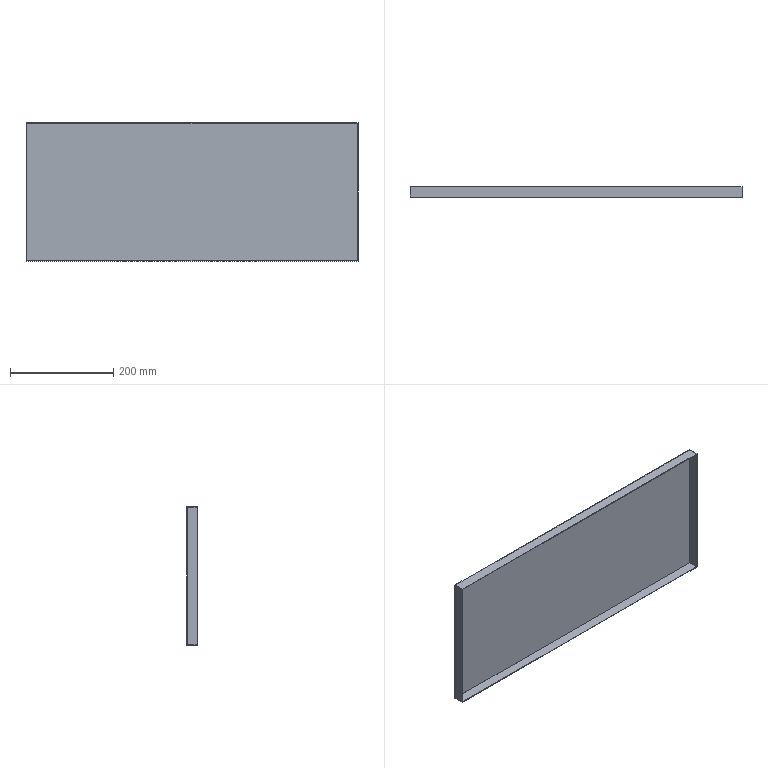Component | SolidWorks | FrameAssembly-1_FrameWeldment-1_BottomThinPlate-1 | 1 solid | 11 faces | box 644 x 20 x 269 mm | volume 248969 mm3 | plane 11
build123d program:
from build123d import *

# Parameters (mm, degrees)
SKETCH1_W           = 644
SKETCH1_H           = 269
BOSS_EXTRUDE1_DEPTH = 20
SKETCH2_W           = 641.6
SKETCH2_H           = 266.6
CUT_EXTRUDE1_DEPTH  = 18.8


with BuildPart() as part:
    # Sketch1 → Boss-Extrude1 (new body)
    with BuildSketch(Plane(origin=(0, 0, 0), x_dir=(-1, 0, 0), z_dir=(0, 0, -1))):
        Rectangle(SKETCH1_W, SKETCH1_H)
    extrude(amount=-BOSS_EXTRUDE1_DEPTH)

    # Sketch2 → Cut-Extrude1 (cut)
    with BuildSketch(Plane(origin=(0, 0, 0), x_dir=(-1, 0, 0), z_dir=(0, 0, -1))):
        Rectangle(SKETCH2_W, SKETCH2_H)
    extrude(amount=-CUT_EXTRUDE1_DEPTH, mode=Mode.SUBTRACT)


solid = part.part

# Placed as in the assembly
solid = solid.moved(Location((-298.746, -418.627, -192), (-90, 0, 0)))
STEP:
#1=COLOUR_RGB('',0.7922,0.8196,0.9333);
#2=FILL_AREA_STYLE_COLOUR('',#1);
#3=FILL_AREA_STYLE('',(#2));
#4=SURFACE_STYLE_FILL_AREA(#3);
#5=SURFACE_SIDE_STYLE('',(#4));
#6=SURFACE_STYLE_USAGE(.BOTH.,#5);
#7=PRESENTATION_STYLE_ASSIGNMENT((#6));
#8=CARTESIAN_POINT('',(0.9155,-16.481,-2.264));
#9=VERTEX_POINT('',#8);
#10=CARTESIAN_POINT('',(-24.439,-16.481,-2.264));
#11=VERTEX_POINT('',#10);
#12=CARTESIAN_POINT('',(0.9155,-16.481,-2.264));
#13=DIRECTION('',(-1.,0.,0.));
#14=VECTOR('',#13,39.37);
#15=LINE('',#12,#14);
#16=EDGE_CURVE('',#9,#11,#15,.T.);
#17=ORIENTED_EDGE('',*,*,#16,.F.);
#18=CARTESIAN_POINT('',(0.9155,-15.694,-2.264));
#19=VERTEX_POINT('',#18);
#20=CARTESIAN_POINT('',(0.9155,-15.694,-2.264));
#21=DIRECTION('',(-0.,-1.,0.));
#22=VECTOR('',#21,39.37);
#23=LINE('',#20,#22);
#24=EDGE_CURVE('',#19,#9,#23,.T.);
#25=ORIENTED_EDGE('',*,*,#24,.F.);
#26=CARTESIAN_POINT('',(-24.439,-15.694,-2.264));
#27=VERTEX_POINT('',#26);
#28=CARTESIAN_POINT('',(0.9155,-15.694,-2.264));
#29=DIRECTION('',(-1.,0.,0.));
#30=VECTOR('',#29,39.37);
#31=LINE('',#28,#30);
#32=EDGE_CURVE('',#19,#27,#31,.T.);
#33=ORIENTED_EDGE('',*,*,#32,.T.);
#34=CARTESIAN_POINT('',(-24.439,-15.694,-2.264));
#35=DIRECTION('',(-0.,-1.,0.));
#36=VECTOR('',#35,39.37);
#37=LINE('',#34,#36);
#38=EDGE_CURVE('',#27,#11,#37,.T.);
#39=ORIENTED_EDGE('',*,*,#38,.T.);
#40=EDGE_LOOP('',(#17,#25,#33,#39));
#41=FACE_OUTER_BOUND('',#40,.T.);
#42=CARTESIAN_POINT('',(0.9155,-15.694,-2.264));
#43=DIRECTION('',(0.,0.,1.));
#44=DIRECTION('',(-0.,-1.,0.));
#45=AXIS2_PLACEMENT_3D('',#42,#43,#44);
#46=PLANE('',#45);
#47=ADVANCED_FACE('',(#41),#46,.T.);
#48=CARTESIAN_POINT('',(0.9155,-16.481,-12.854));
#49=VERTEX_POINT('',#48);
#50=CARTESIAN_POINT('',(0.9155,-16.481,-12.854));
#51=DIRECTION('',(-0.,0.,1.));
#52=VECTOR('',#51,39.37);
#53=LINE('',#50,#52);
#54=EDGE_CURVE('',#49,#9,#53,.T.);
#55=ORIENTED_EDGE('',*,*,#54,.F.);
#56=CARTESIAN_POINT('',(0.9155,-15.694,-12.854));
#57=VERTEX_POINT('',#56);
#58=CARTESIAN_POINT('',(0.9155,-15.694,-12.854));
#59=DIRECTION('',(-0.,-1.,0.));
#60=VECTOR('',#59,39.37);
#61=LINE('',#58,#60);
#62=EDGE_CURVE('',#57,#49,#61,.T.);
#63=ORIENTED_EDGE('',*,*,#62,.F.);
#64=CARTESIAN_POINT('',(0.9155,-15.694,-12.854));
#65=DIRECTION('',(-0.,0.,1.));
#66=VECTOR('',#65,39.37);
#67=LINE('',#64,#66);
#68=EDGE_CURVE('',#57,#19,#67,.T.);
#69=ORIENTED_EDGE('',*,*,#68,.T.);
#70=ORIENTED_EDGE('',*,*,#24,.T.);
#71=EDGE_LOOP('',(#55,#63,#69,#70));
#72=FACE_OUTER_BOUND('',#71,.T.);
#73=CARTESIAN_POINT('',(0.9155,-15.694,-12.854));
#74=DIRECTION('',(1.,-0.,0.));
#75=DIRECTION('',(0.,-0.,-1.));
#76=AXIS2_PLACEMENT_3D('',#73,#74,#75);
#77=PLANE('',#76);
#78=ADVANCED_FACE('',(#72),#77,.T.);
#79=CARTESIAN_POINT('',(-24.439,-16.481,-12.854));
#80=VERTEX_POINT('',#79);
#81=CARTESIAN_POINT('',(-24.439,-16.481,-12.854));
#82=DIRECTION('',(1.,-0.,0.));
#83=VECTOR('',#82,39.37);
#84=LINE('',#81,#83);
#85=EDGE_CURVE('',#80,#49,#84,.T.);
#86=ORIENTED_EDGE('',*,*,#85,.F.);
#87=CARTESIAN_POINT('',(-24.439,-15.694,-12.854));
#88=VERTEX_POINT('',#87);
#89=CARTESIAN_POINT('',(-24.439,-15.694,-12.854));
#90=DIRECTION('',(-0.,-1.,0.));
#91=VECTOR('',#90,39.37);
#92=LINE('',#89,#91);
#93=EDGE_CURVE('',#88,#80,#92,.T.);
#94=ORIENTED_EDGE('',*,*,#93,.F.);
#95=CARTESIAN_POINT('',(-24.439,-15.694,-12.854));
#96=DIRECTION('',(1.,-0.,0.));
#97=VECTOR('',#96,39.37);
#98=LINE('',#95,#97);
#99=EDGE_CURVE('',#88,#57,#98,.T.);
#100=ORIENTED_EDGE('',*,*,#99,.T.);
#101=ORIENTED_EDGE('',*,*,#62,.T.);
#102=EDGE_LOOP('',(#86,#94,#100,#101));
#103=FACE_OUTER_BOUND('',#102,.T.);
#104=CARTESIAN_POINT('',(-24.439,-15.694,-12.854));
#105=DIRECTION('',(-0.,-0.,-1.));
#106=DIRECTION('',(0.,1.,-0.));
#107=AXIS2_PLACEMENT_3D('',#104,#105,#106);
#108=PLANE('',#107);
#109=ADVANCED_FACE('',(#103),#108,.T.);
#110=CARTESIAN_POINT('',(-24.439,-16.481,-2.264));
#111=DIRECTION('',(-0.,0.,-1.));
#112=VECTOR('',#111,39.37);
#113=LINE('',#110,#112);
#114=EDGE_CURVE('',#11,#80,#113,.T.);
#115=ORIENTED_EDGE('',*,*,#114,.F.);
#116=ORIENTED_EDGE('',*,*,#38,.F.);
#117=CARTESIAN_POINT('',(-24.439,-15.694,-2.264));
#118=DIRECTION('',(-0.,0.,-1.));
#119=VECTOR('',#118,39.37);
#120=LINE('',#117,#119);
#121=EDGE_CURVE('',#27,#88,#120,.T.);
#122=ORIENTED_EDGE('',*,*,#121,.T.);
#123=ORIENTED_EDGE('',*,*,#93,.T.);
#124=EDGE_LOOP('',(#115,#116,#122,#123));
#125=FACE_OUTER_BOUND('',#124,.T.);
#126=CARTESIAN_POINT('',(-24.439,-15.694,-2.264));
#127=DIRECTION('',(-1.,0.,0.));
#128=DIRECTION('',(0.,-0.,1.));
#129=AXIS2_PLACEMENT_3D('',#126,#127,#128);
#130=PLANE('',#129);
#131=ADVANCED_FACE('',(#125),#130,.T.);
#132=ORIENTED_EDGE('',*,*,#32,.F.);
#133=ORIENTED_EDGE('',*,*,#68,.F.);
#134=ORIENTED_EDGE('',*,*,#99,.F.);
#135=ORIENTED_EDGE('',*,*,#121,.F.);
#136=EDGE_LOOP('',(#132,#133,#134,#135));
#137=FACE_OUTER_BOUND('',#136,.T.);
#138=CARTESIAN_POINT('',(-11.762,-15.694,-7.559));
#139=DIRECTION('',(-0.,-1.,0.));
#140=DIRECTION('',(-1.,0.,0.));
#141=AXIS2_PLACEMENT_3D('',#138,#139,#140);
#142=PLANE('',#141);
#143=ADVANCED_FACE('',(#137),#142,.F.);
#144=CARTESIAN_POINT('',(0.8683,-16.481,-12.807));
#145=VERTEX_POINT('',#144);
#146=CARTESIAN_POINT('',(0.8683,-16.481,-2.311));
#147=VERTEX_POINT('',#146);
#148=CARTESIAN_POINT('',(0.8683,-16.481,-12.807));
#149=DIRECTION('',(0.,0.,1.));
#150=VECTOR('',#149,39.37);
#151=LINE('',#148,#150);
#152=EDGE_CURVE('',#145,#147,#151,.T.);
#153=ORIENTED_EDGE('',*,*,#152,.F.);
#154=CARTESIAN_POINT('',(-24.392,-16.481,-12.807));
#155=VERTEX_POINT('',#154);
#156=CARTESIAN_POINT('',(-24.392,-16.481,-12.807));
#157=DIRECTION('',(1.,-0.,0.));
#158=VECTOR('',#157,39.37);
#159=LINE('',#156,#158);
#160=EDGE_CURVE('',#155,#145,#159,.T.);
#161=ORIENTED_EDGE('',*,*,#160,.F.);
#162=CARTESIAN_POINT('',(-24.392,-16.481,-2.311));
#163=VERTEX_POINT('',#162);
#164=CARTESIAN_POINT('',(-24.392,-16.481,-2.311));
#165=DIRECTION('',(-0.,-0.,-1.));
#166=VECTOR('',#165,39.37);
#167=LINE('',#164,#166);
#168=EDGE_CURVE('',#163,#155,#167,.T.);
#169=ORIENTED_EDGE('',*,*,#168,.F.);
#170=CARTESIAN_POINT('',(0.8683,-16.481,-2.311));
#171=DIRECTION('',(-1.,0.,0.));
#172=VECTOR('',#171,39.37);
#173=LINE('',#170,#172);
#174=EDGE_CURVE('',#147,#163,#173,.T.);
#175=ORIENTED_EDGE('',*,*,#174,.F.);
#176=EDGE_LOOP('',(#153,#161,#169,#175));
#177=FACE_BOUND('',#176,.T.);
#178=ORIENTED_EDGE('',*,*,#16,.T.);
#179=ORIENTED_EDGE('',*,*,#114,.T.);
#180=ORIENTED_EDGE('',*,*,#85,.T.);
#181=ORIENTED_EDGE('',*,*,#54,.T.);
#182=EDGE_LOOP('',(#178,#179,#180,#181));
#183=FACE_OUTER_BOUND('',#182,.T.);
#184=CARTESIAN_POINT('',(-11.762,-16.481,-7.559));
#185=DIRECTION('',(-0.,-1.,0.));
#186=DIRECTION('',(-1.,0.,0.));
#187=AXIS2_PLACEMENT_3D('',#184,#185,#186);
#188=PLANE('',#187);
#189=ADVANCED_FACE('',(#177,#183),#188,.T.);
#190=ORIENTED_EDGE('',*,*,#152,.T.);
#191=CARTESIAN_POINT('',(0.8683,-15.741,-2.311));
#192=VERTEX_POINT('',#191);
#193=CARTESIAN_POINT('',(0.8683,-15.741,-2.311));
#194=DIRECTION('',(-0.,-1.,0.));
#195=VECTOR('',#194,39.37);
#196=LINE('',#193,#195);
#197=EDGE_CURVE('',#192,#147,#196,.T.);
#198=ORIENTED_EDGE('',*,*,#197,.F.);
#199=CARTESIAN_POINT('',(0.8683,-15.741,-12.807));
#200=VERTEX_POINT('',#199);
#201=CARTESIAN_POINT('',(0.8683,-15.741,-12.807));
#202=DIRECTION('',(0.,0.,1.));
#203=VECTOR('',#202,39.37);
#204=LINE('',#201,#203);
#205=EDGE_CURVE('',#200,#192,#204,.T.);
#206=ORIENTED_EDGE('',*,*,#205,.F.);
#207=CARTESIAN_POINT('',(0.8683,-15.741,-12.807));
#208=DIRECTION('',(-0.,-1.,0.));
#209=VECTOR('',#208,39.37);
#210=LINE('',#207,#209);
#211=EDGE_CURVE('',#200,#145,#210,.T.);
#212=ORIENTED_EDGE('',*,*,#211,.T.);
#213=EDGE_LOOP('',(#190,#198,#206,#212));
#214=FACE_OUTER_BOUND('',#213,.T.);
#215=CARTESIAN_POINT('',(0.8683,-15.741,-12.807));
#216=DIRECTION('',(1.,-0.,0.));
#217=DIRECTION('',(-0.,-1.,0.));
#218=AXIS2_PLACEMENT_3D('',#215,#216,#217);
#219=PLANE('',#218);
#220=ADVANCED_FACE('',(#214),#219,.F.);
#221=ORIENTED_EDGE('',*,*,#160,.T.);
#222=ORIENTED_EDGE('',*,*,#211,.F.);
#223=CARTESIAN_POINT('',(-24.392,-15.741,-12.807));
#224=VERTEX_POINT('',#223);
#225=CARTESIAN_POINT('',(-24.392,-15.741,-12.807));
#226=DIRECTION('',(1.,-0.,0.));
#227=VECTOR('',#226,39.37);
#228=LINE('',#225,#227);
#229=EDGE_CURVE('',#224,#200,#228,.T.);
#230=ORIENTED_EDGE('',*,*,#229,.F.);
#231=CARTESIAN_POINT('',(-24.392,-15.741,-12.807));
#232=DIRECTION('',(-0.,-1.,0.));
#233=VECTOR('',#232,39.37);
#234=LINE('',#231,#233);
#235=EDGE_CURVE('',#224,#155,#234,.T.);
#236=ORIENTED_EDGE('',*,*,#235,.T.);
#237=EDGE_LOOP('',(#221,#222,#230,#236));
#238=FACE_OUTER_BOUND('',#237,.T.);
#239=CARTESIAN_POINT('',(-24.392,-15.741,-12.807));
#240=DIRECTION('',(-0.,-0.,-1.));
#241=DIRECTION('',(0.,1.,-0.));
#242=AXIS2_PLACEMENT_3D('',#239,#240,#241);
#243=PLANE('',#242);
#244=ADVANCED_FACE('',(#238),#243,.F.);
#245=ORIENTED_EDGE('',*,*,#168,.T.);
#246=ORIENTED_EDGE('',*,*,#235,.F.);
#247=CARTESIAN_POINT('',(-24.392,-15.741,-2.311));
#248=VERTEX_POINT('',#247);
#249=CARTESIAN_POINT('',(-24.392,-15.741,-2.311));
#250=DIRECTION('',(-0.,-0.,-1.));
#251=VECTOR('',#250,39.37);
#252=LINE('',#249,#251);
#253=EDGE_CURVE('',#248,#224,#252,.T.);
#254=ORIENTED_EDGE('',*,*,#253,.F.);
#255=CARTESIAN_POINT('',(-24.392,-15.741,-2.311));
#256=DIRECTION('',(-0.,-1.,0.));
#257=VECTOR('',#256,39.37);
#258=LINE('',#255,#257);
#259=EDGE_CURVE('',#248,#163,#258,.T.);
#260=ORIENTED_EDGE('',*,*,#259,.T.);
#261=EDGE_LOOP('',(#245,#246,#254,#260));
#262=FACE_OUTER_BOUND('',#261,.T.);
#263=CARTESIAN_POINT('',(-24.392,-15.741,-2.311));
#264=DIRECTION('',(-1.,0.,-0.));
#265=DIRECTION('',(0.,1.,-0.));
#266=AXIS2_PLACEMENT_3D('',#263,#264,#265);
#267=PLANE('',#266);
#268=ADVANCED_FACE('',(#262),#267,.F.);
#269=ORIENTED_EDGE('',*,*,#174,.T.);
#270=ORIENTED_EDGE('',*,*,#259,.F.);
#271=CARTESIAN_POINT('',(0.8683,-15.741,-2.311));
#272=DIRECTION('',(-1.,0.,0.));
#273=VECTOR('',#272,39.37);
#274=LINE('',#271,#273);
#275=EDGE_CURVE('',#192,#248,#274,.T.);
#276=ORIENTED_EDGE('',*,*,#275,.F.);
#277=ORIENTED_EDGE('',*,*,#197,.T.);
#278=EDGE_LOOP('',(#269,#270,#276,#277));
#279=FACE_OUTER_BOUND('',#278,.T.);
#280=CARTESIAN_POINT('',(0.8683,-15.741,-2.311));
#281=DIRECTION('',(0.,0.,1.));
#282=DIRECTION('',(-0.,-1.,0.));
#283=AXIS2_PLACEMENT_3D('',#280,#281,#282);
#284=PLANE('',#283);
#285=ADVANCED_FACE('',(#279),#284,.F.);
#286=ORIENTED_EDGE('',*,*,#205,.T.);
#287=ORIENTED_EDGE('',*,*,#275,.T.);
#288=ORIENTED_EDGE('',*,*,#253,.T.);
#289=ORIENTED_EDGE('',*,*,#229,.T.);
#290=EDGE_LOOP('',(#286,#287,#288,#289));
#291=FACE_OUTER_BOUND('',#290,.T.);
#292=CARTESIAN_POINT('',(-11.762,-15.741,-7.559));
#293=DIRECTION('',(-0.,-1.,0.));
#294=DIRECTION('',(-1.,0.,0.));
#295=AXIS2_PLACEMENT_3D('',#292,#293,#294);
#296=PLANE('',#295);
#297=ADVANCED_FACE('',(#291),#296,.T.);
#298=CLOSED_SHELL('',(#47,#78,#109,#131,#143,#189,#220,#244,#268,#285,#297));
#299=MANIFOLD_SOLID_BREP('',#298);
#300=STYLED_ITEM('',(#7),#299);
#301=(LENGTH_UNIT()NAMED_UNIT(*)SI_UNIT($,.METRE.));
#302=LENGTH_MEASURE_WITH_UNIT(LENGTH_MEASURE(0.0254),#301);
#303=DIMENSIONAL_EXPONENTS(1.,0.,0.,0.,0.,0.,0.);
#304=(CONVERSION_BASED_UNIT('',#302)LENGTH_UNIT()NAMED_UNIT(#303));
#305=UNCERTAINTY_MEASURE_WITH_UNIT(LENGTH_MEASURE(0.00001),#304,'','');
#306=(NAMED_UNIT(*)PLANE_ANGLE_UNIT()SI_UNIT($,.RADIAN.));
#307=(NAMED_UNIT(*)SI_UNIT($,.STERADIAN.)SOLID_ANGLE_UNIT());
#308=(GEOMETRIC_REPRESENTATION_CONTEXT(3)GLOBAL_UNCERTAINTY_ASSIGNED_CONTEXT((#305))GLOBAL_UNIT_ASSIGNED_CONTEXT((#304,#306,#307))REPRESENTATION_CONTEXT('',''));
#309=MECHANICAL_DESIGN_GEOMETRIC_PRESENTATION_REPRESENTATION('',(#300),#308);
#310=CARTESIAN_POINT('',(0.,0.,0.));
#311=DIRECTION('',(0.,0.,1.));
#312=DIRECTION('',(1.,0.,0.));
#313=AXIS2_PLACEMENT_3D('',#310,#311,#312);
#314=(LENGTH_UNIT()NAMED_UNIT(*)SI_UNIT($,.METRE.));
#315=LENGTH_MEASURE_WITH_UNIT(LENGTH_MEASURE(0.0254),#314);
#316=DIMENSIONAL_EXPONENTS(1.,0.,0.,0.,0.,0.,0.);
#317=(CONVERSION_BASED_UNIT('',#315)LENGTH_UNIT()NAMED_UNIT(#316));
#318=UNCERTAINTY_MEASURE_WITH_UNIT(LENGTH_MEASURE(0.00001),#317,'','');
#319=(NAMED_UNIT(*)PLANE_ANGLE_UNIT()SI_UNIT($,.RADIAN.));
#320=(NAMED_UNIT(*)SI_UNIT($,.STERADIAN.)SOLID_ANGLE_UNIT());
#321=(GEOMETRIC_REPRESENTATION_CONTEXT(3)GLOBAL_UNCERTAINTY_ASSIGNED_CONTEXT((#318))GLOBAL_UNIT_ASSIGNED_CONTEXT((#317,#319,#320))REPRESENTATION_CONTEXT('',''));
#322=ADVANCED_BREP_SHAPE_REPRESENTATION('',(#299,#313),#321);
#323=PRESENTATION_LAYER_ASSIGNMENT('','',(#300));